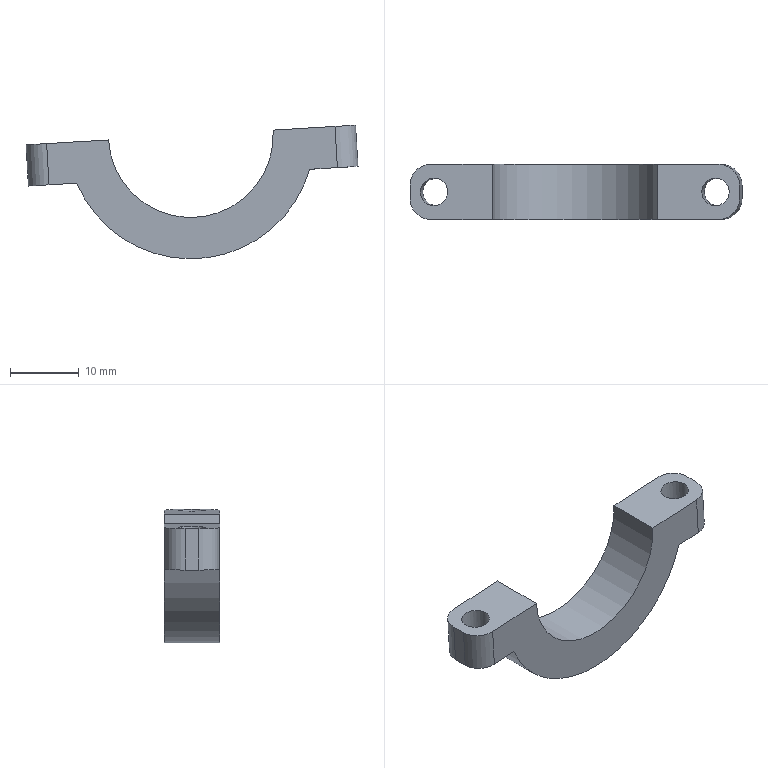Component | NX | LOWER_PISTON_CONNECTING_ROD | 1 solid | 16 faces | volume 2673 mm3 | plane 8 | cylinder 8 | commonest cylinder face diameters 6 x4 4 x2 36 x1 24 x1